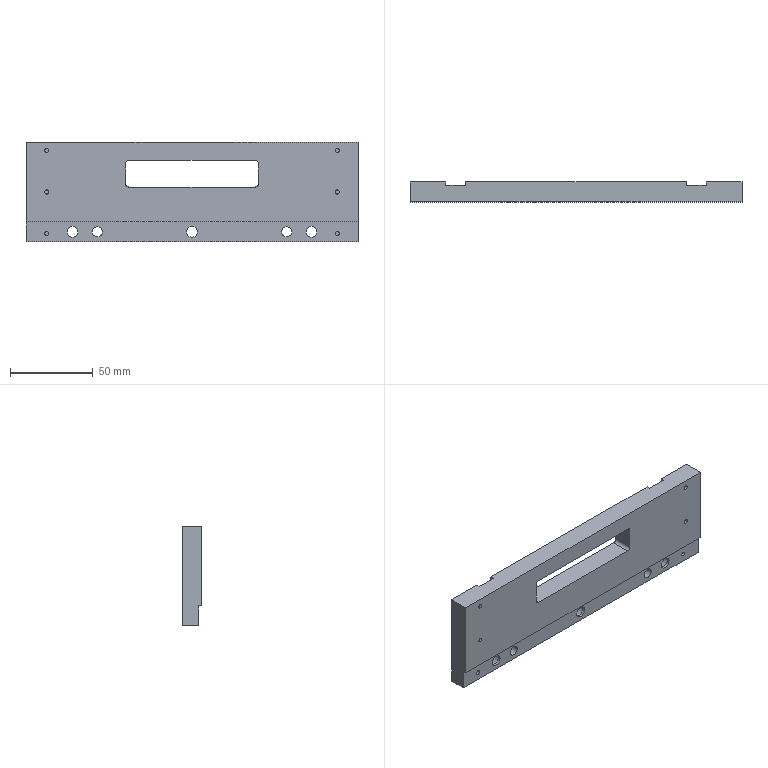Component | SolidWorks | 12-DividingMechanism-1111-1_13-1111-1 | 1 solid | 67 faces | box 200 x 12 x 60 mm | volume 112981 mm3 | cylinder 34 | plane 33 | commonest cylinder face diameters 2.5 x12 6.6 x6 11 x6 4 x6 6 x4
build123d program:
from build123d import *

# Parameters (mm, degrees)
SKETCH5_W                                       = 60
SKETCH5_H                                       = 200
BOSS_EXTRUDE1_DEPTH                             = 12
SKETCH6_W                                       = 60
SKETCH6_H                                       = 12
CUT_EXTRUDE1_DEPTH                              = 2
SKETCH33_W                                      = 12
SKETCH33_H                                      = 200
CUT_EXTRUDE5_DEPTH                              = 2
SKETCH34_W                                      = 16
SKETCH34_H                                      = 80
CUT_EXTRUDE6_DEPTH                              = 106.09
FILLET4_R                                       = 2
CUT_EXTRUDE7_DEPTH                              = 2.5
SKETCH37_W                                      = 1.25
SKETCH37_H                                      = 10
M3_TAPPED_HOLE2_AT_2_COUNT                      = 2
M3_TAPPED_HOLE2_AT_2_PITCH                      = 25
M3_TAPPED_HOLE2_AT_3_COUNT                      = 2
M3_TAPPED_HOLE2_AT_3_PITCH                      = 50
MIRROR2_COPY_1_SKETCH_W                         = 1.25
MIRROR2_COPY_1_SKETCH_H                         = 10
MIRROR2_COPY_2_SKETCH_W                         = 1.25
MIRROR2_COPY_2_SKETCH_H                         = 10
M6_HEX_SOCKET_HEAD_CAP_SCREW_CBORE1_D           = 6.6
M6_HEX_SOCKET_HEAD_CAP_SCREW_CBORE1_CBORE_D     = 11
M6_HEX_SOCKET_HEAD_CAP_SCREW_CBORE1_CBORE_DEPTH = 8.5
SIZE_MM_DOWEL_PIN_HOLE0_D                       = 6


with BuildPart() as part:
    # Sketch5 → Boss-Extrude1 (new body)
    with BuildSketch(Plane(origin=(0, 0, 0), x_dir=(1, 0, 0), z_dir=(0, 1, 0))):
        Rectangle(SKETCH5_W, SKETCH5_H)
    extrude(amount=BOSS_EXTRUDE1_DEPTH)

    # Sketch6 → Cut-Extrude1 (cut)
    with BuildSketch(Plane(origin=(0, 12, 0), x_dir=(1, 0, 0), z_dir=(0, 1, 0))):
        with Locations((0, -72.5)):
            Rectangle(SKETCH6_W, SKETCH6_H)
        with Locations((0, 72.5)):
            Rectangle(SKETCH6_W, SKETCH6_H)
    extrude(amount=-CUT_EXTRUDE1_DEPTH, mode=Mode.SUBTRACT)

    # Sketch33 → Cut-Extrude5 (cut)
    with BuildSketch(Plane.XZ):
        with Locations((-24, 0)):
            Rectangle(SKETCH33_W, SKETCH33_H)
    extrude(amount=-CUT_EXTRUDE5_DEPTH, mode=Mode.SUBTRACT)

    # Sketch34 → Cut-Extrude6 (cut, through all)
    with BuildSketch(Plane.XZ):
        with Locations((11, 0)):
            Rectangle(SKETCH34_W, SKETCH34_H)
    extrude(amount=-CUT_EXTRUDE6_DEPTH, mode=Mode.SUBTRACT)

    # Fillet4
    fillet4_edges = [part.edges().sort_by_distance(p)[0] for p in [
        (3, 6, -40),
        (3, 6, 40),
        (19, 6, 40),
        (19, 6, -40),
    ]]
    fillet(fillet4_edges, radius=FILLET4_R)

    # Sketch35 → Cut-Extrude7 (cut)
    with BuildSketch(Plane(origin=(0, 12, 0), x_dir=(1, 0, 0), z_dir=(0, 1, 0))):
        with BuildLine():
            Line((-8, -45.5), (-8, 45.5))
            ThreePointArc((-8, 45.5), (-8.586, 46.914), (-10, 47.5))
            Line((-10, 47.5), (-30, 47.5))
            Line((-30, 47.5), (-30, -47.5))
            Line((-30, -47.5), (-10, -47.5))
            ThreePointArc((-10, -47.5), (-8.586, -46.914), (-8, -45.5))
        make_face()
    extrude(amount=-CUT_EXTRUDE7_DEPTH, mode=Mode.SUBTRACT)

    # Sketch37 → M3 Tapped Hole2 (revolve, cut)
    with BuildSketch(Plane(origin=(-25, 10, 87.5), x_dir=(0, 0, 1), z_dir=(1, 0, 0))):
        with Locations((0.625, 5)):
            Rectangle(SKETCH37_W, SKETCH37_H)
    m3_tapped_hole2 = revolve(axis=Axis((-25, 16.35, 87.5), (0, -1, 0)), mode=Mode.SUBTRACT)

    # M3 Tapped Hole2 at 2: M3 Tapped Hole2 ×2
    with Locations(*[(i * M3_TAPPED_HOLE2_AT_2_PITCH, 0, 0) for i in range(1, M3_TAPPED_HOLE2_AT_2_COUNT)]):
        add(m3_tapped_hole2, mode=Mode.SUBTRACT)

    # M3 Tapped Hole2 at 3: M3 Tapped Hole2 ×2
    with Locations(*[(i * M3_TAPPED_HOLE2_AT_3_PITCH, 0, 0) for i in range(1, M3_TAPPED_HOLE2_AT_3_COUNT)]):
        add(m3_tapped_hole2, mode=Mode.SUBTRACT)

    # Mirror2: M3 Tapped Hole2 across plane
    add(m3_tapped_hole2.mirror(Plane.XY), mode=Mode.SUBTRACT)

    # Mirror2 copy 1 sketch → Mirror2 copy 1 (revolve, cut)
    with BuildSketch(Plane(origin=(0, 10, -87.5), x_dir=(0, 0, -1), z_dir=(1, 0, 0))):
        with Locations((0.625, -5)):
            Rectangle(MIRROR2_COPY_1_SKETCH_W, MIRROR2_COPY_1_SKETCH_H)
    revolve(axis=Axis((0, 16.35, -87.5), (0, 1, 0)), mode=Mode.SUBTRACT)

    # Mirror2 copy 2 sketch → Mirror2 copy 2 (revolve, cut)
    with BuildSketch(Plane(origin=(25, 10, -87.5), x_dir=(0, 0, -1), z_dir=(1, 0, 0))):
        with Locations((0.625, -5)):
            Rectangle(MIRROR2_COPY_2_SKETCH_W, MIRROR2_COPY_2_SKETCH_H)
    revolve(axis=Axis((25, 16.35, -87.5), (0, 1, 0)), mode=Mode.SUBTRACT)

    # M6 Hex Socket Head Cap Screw CBORE1 (through all)
    with Locations(Plane(origin=(0, 12, 0), x_dir=(1, 0, 0), z_dir=(0, 1, 0))):
        with Locations((-24, 72), (-24, 0), (-24, -72)):
            CounterBoreHole(M6_HEX_SOCKET_HEAD_CAP_SCREW_CBORE1_D / 2, M6_HEX_SOCKET_HEAD_CAP_SCREW_CBORE1_CBORE_D / 2, M6_HEX_SOCKET_HEAD_CAP_SCREW_CBORE1_CBORE_DEPTH)

    # Size mm Dowel Pin Hole0 (through all)
    with Locations(Plane(origin=(0, 12, 0), x_dir=(1, 0, 0), z_dir=(0, 1, 0))):
        with Locations((-24, 57), (-24, -57)):
            Hole(SIZE_MM_DOWEL_PIN_HOLE0_D / 2)


solid = part.part

# Placed as in the assembly
solid = solid.moved(Location((3.428, 539.224, 1534.056), (0, -90, 0)))